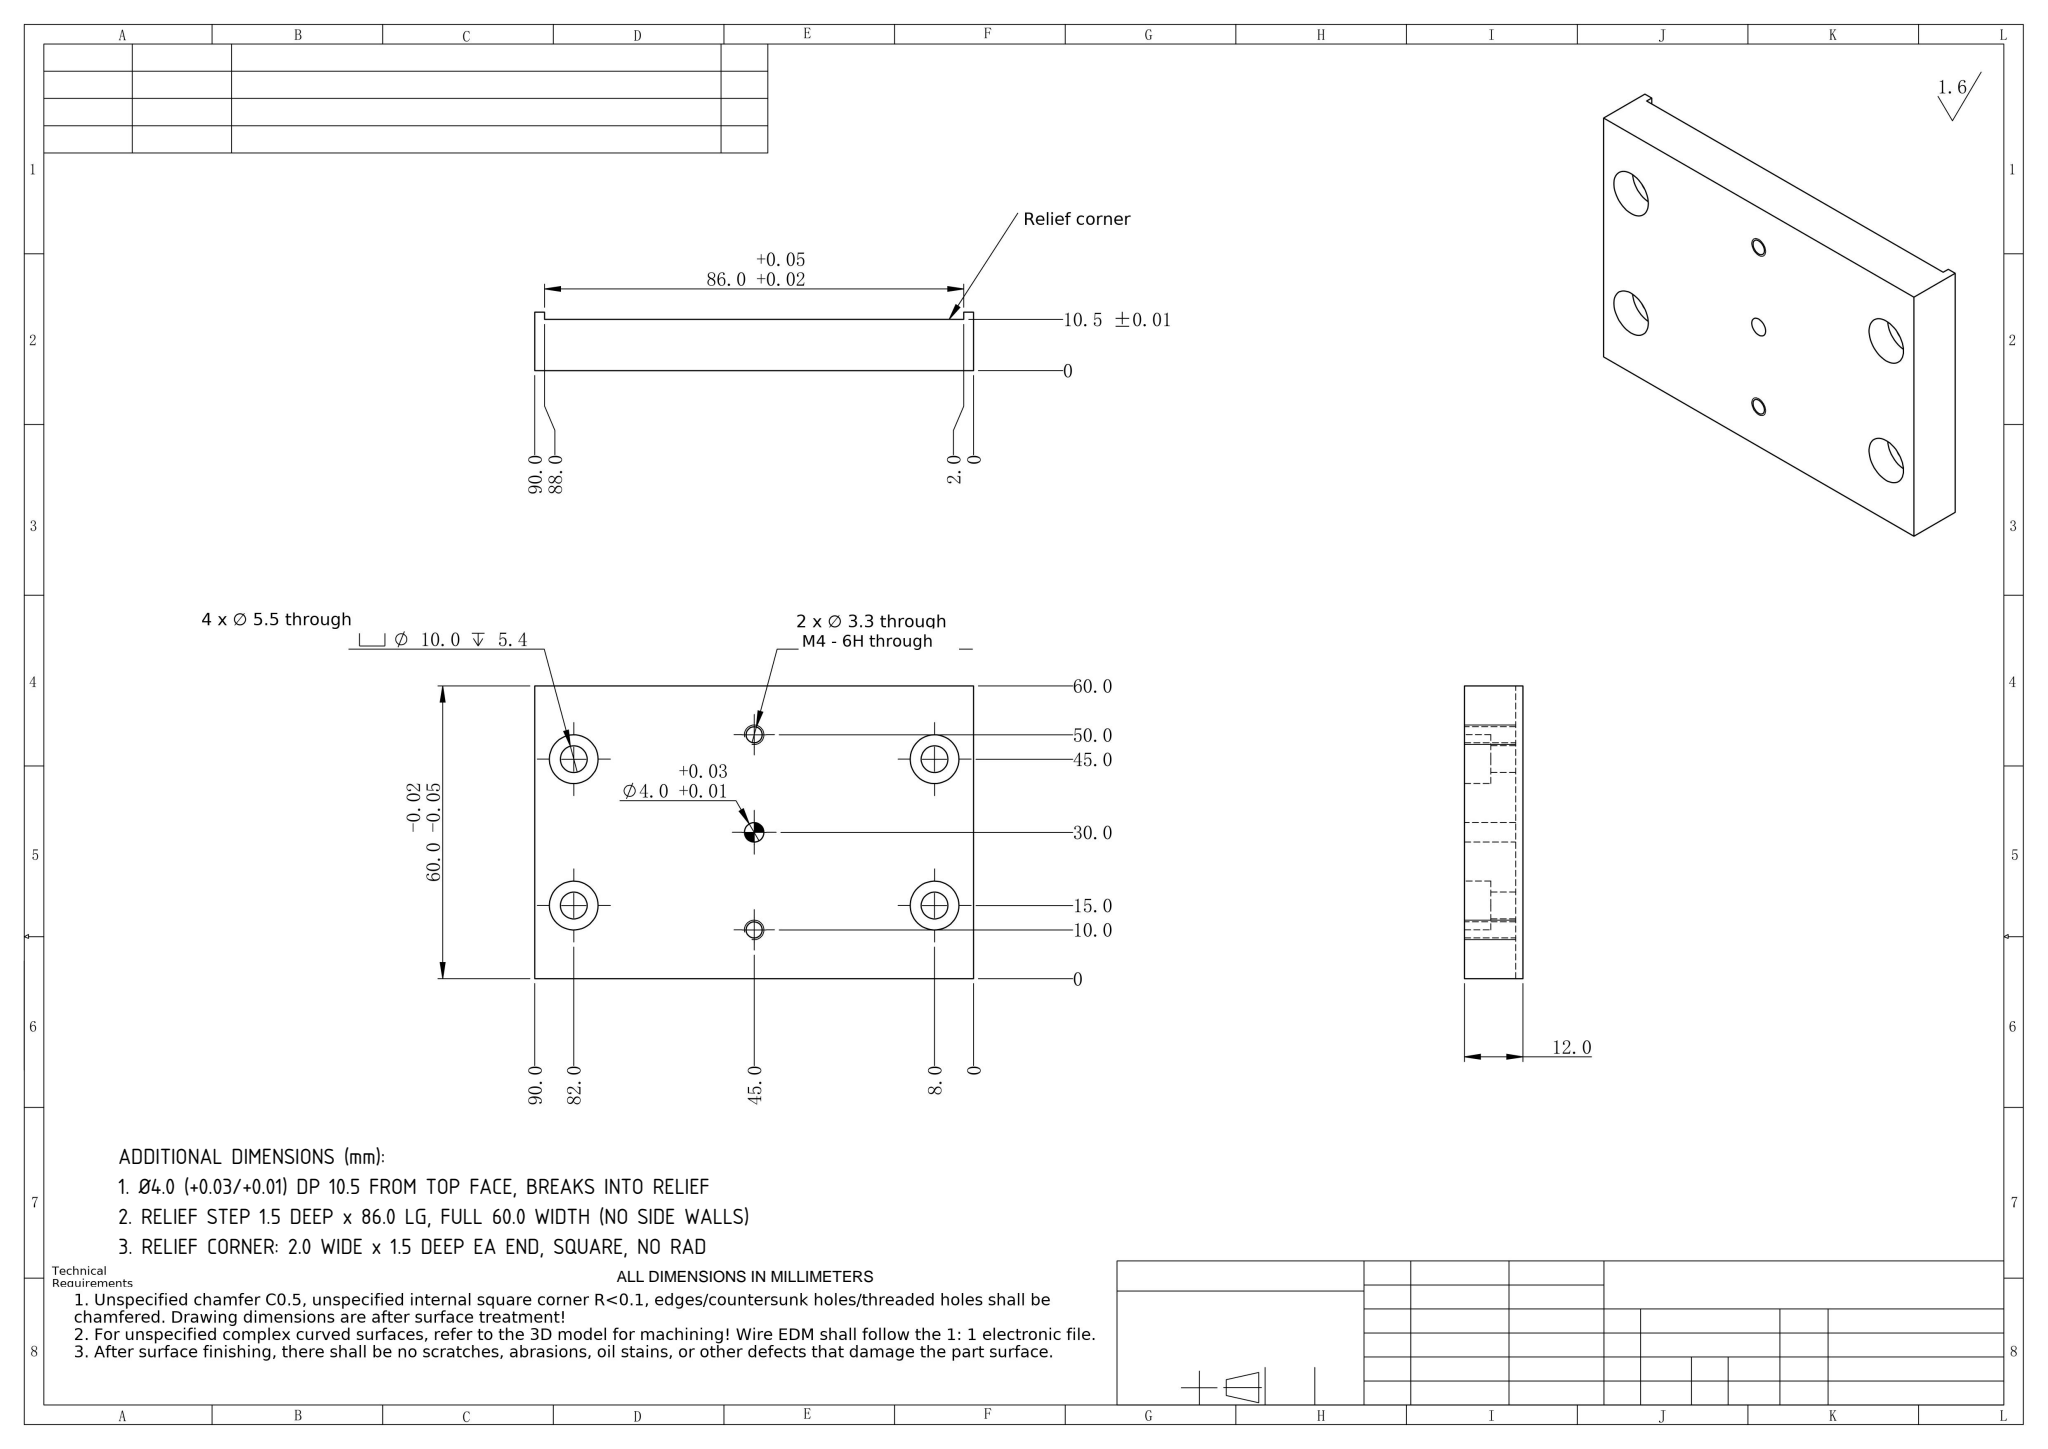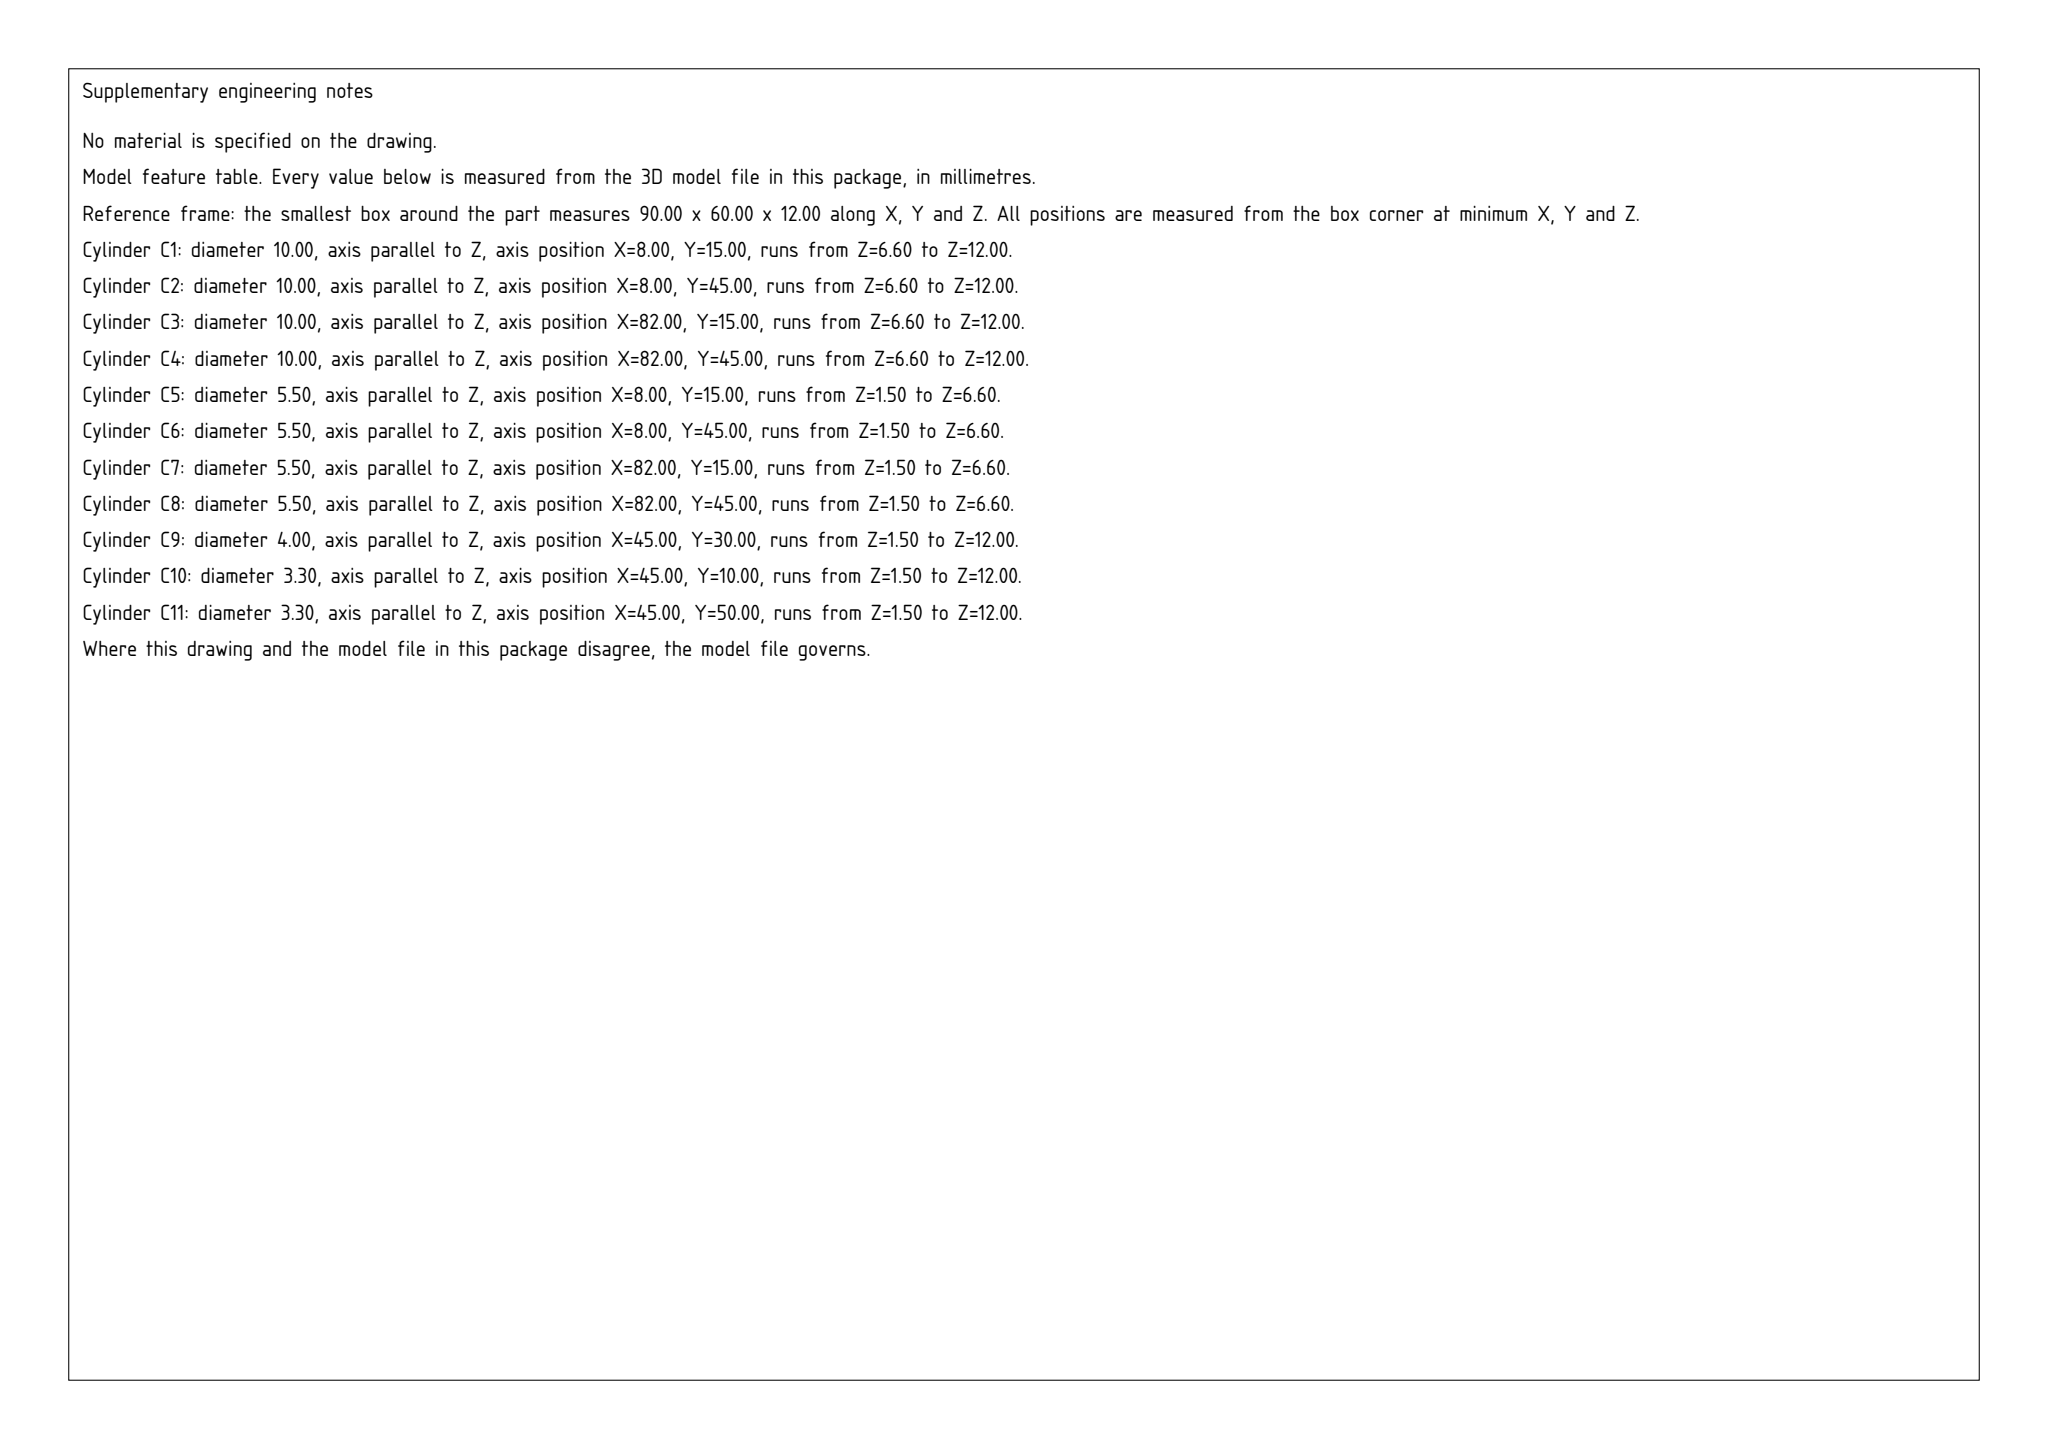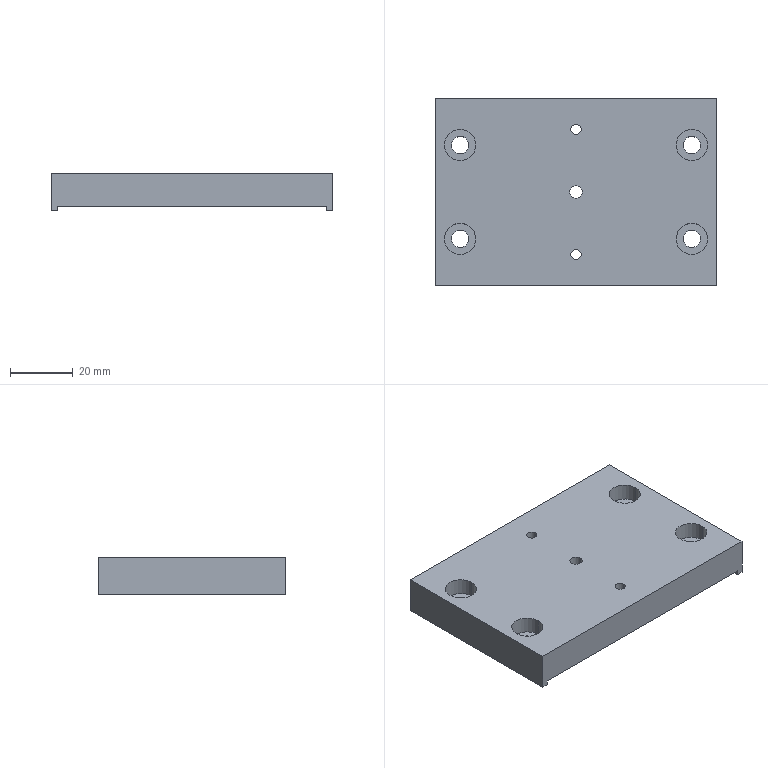Part | SolidWorks | mm | 1 solid | 36 faces | box 90 x 60 x 12 mm | volume 54567 mm3 | cylinder 22 | plane 14 | commonest cylinder face diameters 10 x8 5.5 x8 3.3 x4 4 x2
build123d program:
from build123d import *

# Parameters (mm, degrees)
SKETCH1_W                                       = 90
SKETCH1_H                                       = 60
BOSS_EXTRUDE1_DEPTH                             = 12
SKETCH2_W                                       = 86
SKETCH2_H                                       = 1.5
CUT_EXTRUDE1_DEPTH                              = 109.83
M5_HEX_SOCKET_HEAD_CAP_SCREW_CBORE1_D           = 5.5
M5_HEX_SOCKET_HEAD_CAP_SCREW_CBORE1_CBORE_D     = 10
M5_HEX_SOCKET_HEAD_CAP_SCREW_CBORE1_CBORE_DEPTH = 5.4
M4_TAPPED_HOLE1_D                               = 3.3
SKETCH7_R                                       = 2
CUT_EXTRUDE2_DEPTH                              = 109.83


with BuildPart() as part:
    # Sketch1 → Boss-Extrude1 (new body)
    with BuildSketch(Plane.XY):
        with Locations((45, 30)):
            Rectangle(SKETCH1_W, SKETCH1_H)
    extrude(amount=BOSS_EXTRUDE1_DEPTH)

    # Sketch2 → Cut-Extrude1 (cut, through all)
    with BuildSketch(Plane(origin=(0, 60, 0), x_dir=(1, 0, 0), z_dir=(0, 1, 0))):
        with Locations((45, -0.75)):
            Rectangle(SKETCH2_W, SKETCH2_H)
    extrude(amount=-CUT_EXTRUDE1_DEPTH, mode=Mode.SUBTRACT)

    # M5 Hex Socket Head Cap Screw CBORE1 (through all)
    with Locations(Plane.XY.offset(12)):
        with Locations((8, 45), (8, 15), (82, 45), (82, 15)):
            CounterBoreHole(M5_HEX_SOCKET_HEAD_CAP_SCREW_CBORE1_D / 2, M5_HEX_SOCKET_HEAD_CAP_SCREW_CBORE1_CBORE_D / 2, M5_HEX_SOCKET_HEAD_CAP_SCREW_CBORE1_CBORE_DEPTH)

    # M4 Tapped Hole1 (through all)
    with Locations(Plane.XY.offset(12)):
        with Locations((45, 50), (45, 10)):
            Hole(M4_TAPPED_HOLE1_D / 2)

    # Sketch7 → Cut-Extrude2 (cut, through all)
    with BuildSketch(Plane.XY.offset(12)):
        with Locations((45, 30)):
            Circle(SKETCH7_R)
    extrude(amount=-CUT_EXTRUDE2_DEPTH, mode=Mode.SUBTRACT)


solid = part.part